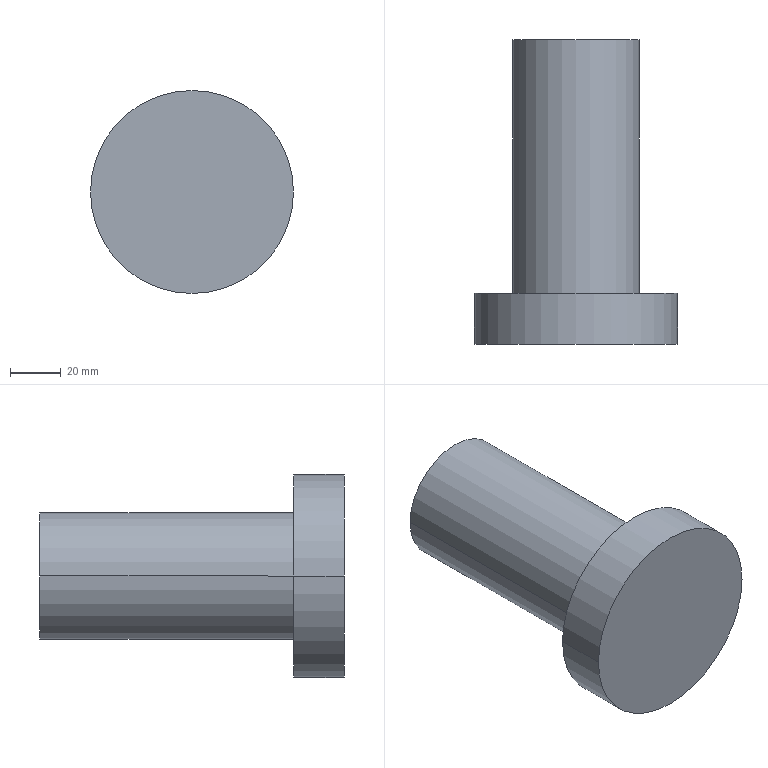Component | SolidWorks | FixedAxis-2 | 1 solid | 7 faces | box 80 x 120 x 80 mm | volume 296881 mm3 | cylinder 4 | plane 3 | commonest cylinder face diameters 80 x2 50 x2
build123d program:
from build123d import *

# Parameters (mm, degrees)
SKETCH1_R           = 25
BOSS_EXTRUDE1_DEPTH = 100
SKETCH3_R           = 40
BOSS_EXTRUDE2_DEPTH = 20


with BuildPart() as part:
    # Sketch1 → Boss-Extrude1 (new body)
    with BuildSketch(Plane.XY):
        with Locations((327.615, 384.486)):
            Circle(SKETCH1_R)
    extrude(amount=-BOSS_EXTRUDE1_DEPTH)

    # Sketch3 → Boss-Extrude2 (add)
    with BuildSketch(Plane.XY):
        with Locations((327.615, 384.486)):
            Circle(SKETCH3_R)
    extrude(amount=BOSS_EXTRUDE2_DEPTH)


solid = part.part

# Placed as in the assembly
solid = solid.moved(Location((-646.586, -831, -723.781), (90, 0, 0)))
STEP:
#1=COLOUR_RGB('',0.7922,0.8196,0.9333);
#2=FILL_AREA_STYLE_COLOUR('',#1);
#3=FILL_AREA_STYLE('',(#2));
#4=SURFACE_STYLE_FILL_AREA(#3);
#5=SURFACE_SIDE_STYLE('',(#4));
#6=SURFACE_STYLE_USAGE(.BOTH.,#5);
#7=PRESENTATION_STYLE_ASSIGNMENT((#6));
#8=CARTESIAN_POINT('',(-14.133,-33.504,-13.358));
#9=VERTEX_POINT('',#8);
#10=CARTESIAN_POINT('',(-10.983,-33.504,-13.358));
#11=VERTEX_POINT('',#10);
#12=CARTESIAN_POINT('',(-12.558,-33.504,-13.358));
#13=DIRECTION('',(-0.,-1.,-0.));
#14=DIRECTION('',(-1.,0.,0.));
#15=AXIS2_PLACEMENT_3D('',#12,#13,#14);
#16=CIRCLE('',#15,1.575);
#17=EDGE_CURVE('',#9,#11,#16,.T.);
#18=ORIENTED_EDGE('',*,*,#17,.F.);
#19=CARTESIAN_POINT('',(-14.133,-32.717,-13.358));
#20=VERTEX_POINT('',#19);
#21=CARTESIAN_POINT('',(-14.133,-33.504,-13.358));
#22=DIRECTION('',(0.,1.,0.));
#23=VECTOR('',#22,39.37);
#24=LINE('',#21,#23);
#25=EDGE_CURVE('',#9,#20,#24,.T.);
#26=ORIENTED_EDGE('',*,*,#25,.T.);
#27=CARTESIAN_POINT('',(-10.983,-32.717,-13.358));
#28=VERTEX_POINT('',#27);
#29=CARTESIAN_POINT('',(-12.558,-32.717,-13.358));
#30=DIRECTION('',(-0.,-1.,-0.));
#31=DIRECTION('',(-1.,0.,0.));
#32=AXIS2_PLACEMENT_3D('',#29,#30,#31);
#33=CIRCLE('',#32,1.575);
#34=EDGE_CURVE('',#20,#28,#33,.T.);
#35=ORIENTED_EDGE('',*,*,#34,.T.);
#36=CARTESIAN_POINT('',(-10.983,-33.504,-13.358));
#37=DIRECTION('',(0.,1.,0.));
#38=VECTOR('',#37,39.37);
#39=LINE('',#36,#38);
#40=EDGE_CURVE('',#11,#28,#39,.T.);
#41=ORIENTED_EDGE('',*,*,#40,.F.);
#42=EDGE_LOOP('',(#18,#26,#35,#41));
#43=FACE_OUTER_BOUND('',#42,.T.);
#44=CARTESIAN_POINT('',(-12.558,-33.504,-13.358));
#45=DIRECTION('',(0.,1.,0.));
#46=DIRECTION('',(1.,0.,0.));
#47=AXIS2_PLACEMENT_3D('',#44,#45,#46);
#48=CYLINDRICAL_SURFACE('',#47,1.575);
#49=ADVANCED_FACE('',(#43),#48,.T.);
#50=CARTESIAN_POINT('',(-13.542,-28.78,-13.358));
#51=VERTEX_POINT('',#50);
#52=CARTESIAN_POINT('',(-11.574,-28.78,-13.358));
#53=VERTEX_POINT('',#52);
#54=CARTESIAN_POINT('',(-12.558,-28.78,-13.358));
#55=DIRECTION('',(-0.,-1.,-0.));
#56=DIRECTION('',(-1.,0.,0.));
#57=AXIS2_PLACEMENT_3D('',#54,#55,#56);
#58=CIRCLE('',#57,0.9843);
#59=EDGE_CURVE('',#51,#53,#58,.T.);
#60=ORIENTED_EDGE('',*,*,#59,.T.);
#61=CARTESIAN_POINT('',(-11.574,-32.717,-13.358));
#62=VERTEX_POINT('',#61);
#63=CARTESIAN_POINT('',(-11.574,-28.78,-13.358));
#64=DIRECTION('',(-0.,-1.,-0.));
#65=VECTOR('',#64,39.37);
#66=LINE('',#63,#65);
#67=EDGE_CURVE('',#53,#62,#66,.T.);
#68=ORIENTED_EDGE('',*,*,#67,.T.);
#69=CARTESIAN_POINT('',(-13.542,-32.717,-13.358));
#70=VERTEX_POINT('',#69);
#71=CARTESIAN_POINT('',(-12.558,-32.717,-13.358));
#72=DIRECTION('',(-0.,-1.,-0.));
#73=DIRECTION('',(-1.,0.,0.));
#74=AXIS2_PLACEMENT_3D('',#71,#72,#73);
#75=CIRCLE('',#74,0.9843);
#76=EDGE_CURVE('',#70,#62,#75,.T.);
#77=ORIENTED_EDGE('',*,*,#76,.F.);
#78=CARTESIAN_POINT('',(-13.542,-28.78,-13.358));
#79=DIRECTION('',(-0.,-1.,-0.));
#80=VECTOR('',#79,39.37);
#81=LINE('',#78,#80);
#82=EDGE_CURVE('',#51,#70,#81,.T.);
#83=ORIENTED_EDGE('',*,*,#82,.F.);
#84=EDGE_LOOP('',(#60,#68,#77,#83));
#85=FACE_OUTER_BOUND('',#84,.T.);
#86=CARTESIAN_POINT('',(-12.558,-28.78,-13.358));
#87=DIRECTION('',(-0.,-1.,-0.));
#88=DIRECTION('',(-1.,0.,0.));
#89=AXIS2_PLACEMENT_3D('',#86,#87,#88);
#90=CYLINDRICAL_SURFACE('',#89,0.9843);
#91=ADVANCED_FACE('',(#85),#90,.T.);
#92=ORIENTED_EDGE('',*,*,#67,.F.);
#93=CARTESIAN_POINT('',(-12.558,-28.78,-13.358));
#94=DIRECTION('',(-0.,-1.,-0.));
#95=DIRECTION('',(-1.,0.,0.));
#96=AXIS2_PLACEMENT_3D('',#93,#94,#95);
#97=CIRCLE('',#96,0.9843);
#98=EDGE_CURVE('',#53,#51,#97,.T.);
#99=ORIENTED_EDGE('',*,*,#98,.T.);
#100=ORIENTED_EDGE('',*,*,#82,.T.);
#101=CARTESIAN_POINT('',(-12.558,-32.717,-13.358));
#102=DIRECTION('',(-0.,-1.,-0.));
#103=DIRECTION('',(-1.,0.,0.));
#104=AXIS2_PLACEMENT_3D('',#101,#102,#103);
#105=CIRCLE('',#104,0.9843);
#106=EDGE_CURVE('',#62,#70,#105,.T.);
#107=ORIENTED_EDGE('',*,*,#106,.F.);
#108=EDGE_LOOP('',(#92,#99,#100,#107));
#109=FACE_OUTER_BOUND('',#108,.T.);
#110=CARTESIAN_POINT('',(-12.558,-28.78,-13.358));
#111=DIRECTION('',(-0.,-1.,-0.));
#112=DIRECTION('',(-1.,0.,0.));
#113=AXIS2_PLACEMENT_3D('',#110,#111,#112);
#114=CYLINDRICAL_SURFACE('',#113,0.9843);
#115=ADVANCED_FACE('',(#109),#114,.T.);
#116=ORIENTED_EDGE('',*,*,#59,.F.);
#117=ORIENTED_EDGE('',*,*,#98,.F.);
#118=EDGE_LOOP('',(#116,#117));
#119=FACE_OUTER_BOUND('',#118,.T.);
#120=CARTESIAN_POINT('',(-12.558,-28.78,-13.358));
#121=DIRECTION('',(-0.,-1.,-0.));
#122=DIRECTION('',(-1.,0.,0.));
#123=AXIS2_PLACEMENT_3D('',#120,#121,#122);
#124=PLANE('',#123);
#125=ADVANCED_FACE('',(#119),#124,.F.);
#126=ORIENTED_EDGE('',*,*,#25,.F.);
#127=CARTESIAN_POINT('',(-12.558,-33.504,-13.358));
#128=DIRECTION('',(-0.,-1.,-0.));
#129=DIRECTION('',(-1.,0.,0.));
#130=AXIS2_PLACEMENT_3D('',#127,#128,#129);
#131=CIRCLE('',#130,1.575);
#132=EDGE_CURVE('',#11,#9,#131,.T.);
#133=ORIENTED_EDGE('',*,*,#132,.F.);
#134=ORIENTED_EDGE('',*,*,#40,.T.);
#135=CARTESIAN_POINT('',(-12.558,-32.717,-13.358));
#136=DIRECTION('',(-0.,-1.,-0.));
#137=DIRECTION('',(-1.,0.,0.));
#138=AXIS2_PLACEMENT_3D('',#135,#136,#137);
#139=CIRCLE('',#138,1.575);
#140=EDGE_CURVE('',#28,#20,#139,.T.);
#141=ORIENTED_EDGE('',*,*,#140,.T.);
#142=EDGE_LOOP('',(#126,#133,#134,#141));
#143=FACE_OUTER_BOUND('',#142,.T.);
#144=CARTESIAN_POINT('',(-12.558,-33.504,-13.358));
#145=DIRECTION('',(0.,1.,0.));
#146=DIRECTION('',(1.,0.,0.));
#147=AXIS2_PLACEMENT_3D('',#144,#145,#146);
#148=CYLINDRICAL_SURFACE('',#147,1.575);
#149=ADVANCED_FACE('',(#143),#148,.T.);
#150=ORIENTED_EDGE('',*,*,#132,.T.);
#151=ORIENTED_EDGE('',*,*,#17,.T.);
#152=EDGE_LOOP('',(#150,#151));
#153=FACE_OUTER_BOUND('',#152,.T.);
#154=CARTESIAN_POINT('',(-12.558,-33.504,-13.358));
#155=DIRECTION('',(-0.,-1.,-0.));
#156=DIRECTION('',(-1.,0.,0.));
#157=AXIS2_PLACEMENT_3D('',#154,#155,#156);
#158=PLANE('',#157);
#159=ADVANCED_FACE('',(#153),#158,.T.);
#160=ORIENTED_EDGE('',*,*,#76,.T.);
#161=ORIENTED_EDGE('',*,*,#106,.T.);
#162=EDGE_LOOP('',(#160,#161));
#163=FACE_BOUND('',#162,.T.);
#164=ORIENTED_EDGE('',*,*,#140,.F.);
#165=ORIENTED_EDGE('',*,*,#34,.F.);
#166=EDGE_LOOP('',(#164,#165));
#167=FACE_OUTER_BOUND('',#166,.T.);
#168=CARTESIAN_POINT('',(-12.558,-32.717,-13.358));
#169=DIRECTION('',(-0.,-1.,-0.));
#170=DIRECTION('',(-1.,0.,0.));
#171=AXIS2_PLACEMENT_3D('',#168,#169,#170);
#172=PLANE('',#171);
#173=ADVANCED_FACE('',(#163,#167),#172,.F.);
#174=CLOSED_SHELL('',(#49,#91,#115,#125,#149,#159,#173));
#175=MANIFOLD_SOLID_BREP('',#174);
#176=STYLED_ITEM('',(#7),#175);
#177=PRESENTATION_LAYER_ASSIGNMENT('','',(#176));
#178=(LENGTH_UNIT()NAMED_UNIT(*)SI_UNIT($,.METRE.));
#179=LENGTH_MEASURE_WITH_UNIT(LENGTH_MEASURE(0.0254),#178);
#180=DIMENSIONAL_EXPONENTS(1.,0.,0.,0.,0.,0.,0.);
#181=(CONVERSION_BASED_UNIT('',#179)LENGTH_UNIT()NAMED_UNIT(#180));
#182=UNCERTAINTY_MEASURE_WITH_UNIT(LENGTH_MEASURE(0.00001),#181,'','');
#183=(NAMED_UNIT(*)PLANE_ANGLE_UNIT()SI_UNIT($,.RADIAN.));
#184=(NAMED_UNIT(*)SI_UNIT($,.STERADIAN.)SOLID_ANGLE_UNIT());
#185=(GEOMETRIC_REPRESENTATION_CONTEXT(3)GLOBAL_UNCERTAINTY_ASSIGNED_CONTEXT((#182))GLOBAL_UNIT_ASSIGNED_CONTEXT((#181,#183,#184))REPRESENTATION_CONTEXT('',''));
#186=MECHANICAL_DESIGN_GEOMETRIC_PRESENTATION_REPRESENTATION('',(#176),#185);
#187=CARTESIAN_POINT('',(0.,0.,0.));
#188=DIRECTION('',(0.,0.,1.));
#189=DIRECTION('',(1.,0.,0.));
#190=AXIS2_PLACEMENT_3D('',#187,#188,#189);
#191=(LENGTH_UNIT()NAMED_UNIT(*)SI_UNIT($,.METRE.));
#192=LENGTH_MEASURE_WITH_UNIT(LENGTH_MEASURE(0.0254),#191);
#193=DIMENSIONAL_EXPONENTS(1.,0.,0.,0.,0.,0.,0.);
#194=(CONVERSION_BASED_UNIT('',#192)LENGTH_UNIT()NAMED_UNIT(#193));
#195=UNCERTAINTY_MEASURE_WITH_UNIT(LENGTH_MEASURE(0.00001),#194,'','');
#196=(NAMED_UNIT(*)PLANE_ANGLE_UNIT()SI_UNIT($,.RADIAN.));
#197=(NAMED_UNIT(*)SI_UNIT($,.STERADIAN.)SOLID_ANGLE_UNIT());
#198=(GEOMETRIC_REPRESENTATION_CONTEXT(3)GLOBAL_UNCERTAINTY_ASSIGNED_CONTEXT((#195))GLOBAL_UNIT_ASSIGNED_CONTEXT((#194,#196,#197))REPRESENTATION_CONTEXT('',''));
#199=ADVANCED_BREP_SHAPE_REPRESENTATION('',(#175,#190),#198);